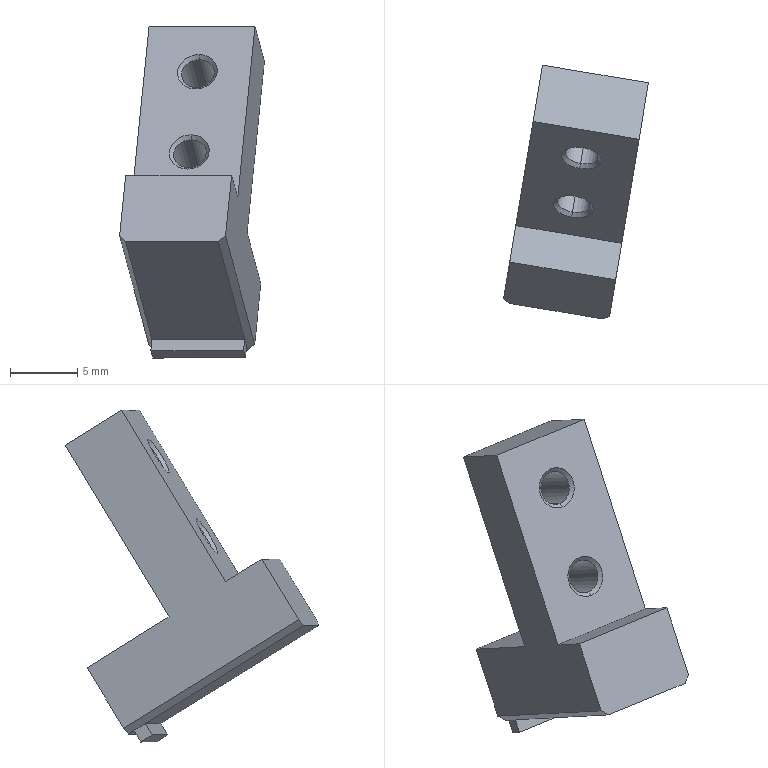Component | SolidWorks | MHZ2_16D_M9BL_14_9_0-1_MHZ2_16D_Finger_0-1 | 1 solid | 30 faces | box 10.79 x 18.88 x 24.73 mm | volume 1274 mm3 | plane 18 | cone 8 | cylinder 4 | commonest cylinder face diameters 2.459 x4
build123d program:
from build123d import *

# Parameters (mm, degrees)
BOSS_EXTRUDE1_DEPTH      = 4
BOSS_EXTRUDE1_DEPTH_BACK = 4
CUT_EXTRUDE1_DEPTH       = 15.5
SKETCH5_W                = 1
SKETCH5_H                = 7
BOSS_EXTRUDE2_DEPTH      = 1


with BuildPart() as part:
    # Sketch1 → Boss-Extrude1 (new, two sides: drawn at the far end of the back side and taken through both)
    with BuildSketch(Plane(origin=(0, 0, 0), x_dir=(1, 0, 0), z_dir=(0, 1, 0)).offset(-BOSS_EXTRUDE1_DEPTH_BACK)):
        Polygon((-18.69, -5.8), (-15.45, -5.8), (-15.45, -20.8), (-10.45, -20.8), (-10.45, -5.8), (-3.19, -5.8), (-3.19, 0), (-18.69, 0), align=None)
    extrude(amount=BOSS_EXTRUDE1_DEPTH + BOSS_EXTRUDE1_DEPTH_BACK)

    # Sketch2 → Cut-Revolve1 (revolve, cut)
    with BuildSketch(Plane(origin=(0, 0, 0), x_dir=(1, 0, 0), z_dir=(0, 1, 0)), mode=Mode.PRIVATE) as cut_revolve1_sk:
        Polygon((-10.45, -16.8), (-10.45, -18.3), (-10.72, -18.029), (-15.18, -18.029), (-15.45, -18.3), (-15.45, -16.8), align=None)
    revolve(cut_revolve1_sk.sketch.rotate(Axis((-15.45, 0, 16.8), (1, 0, 0)), 180), axis=Axis((-15.45, 0, 16.8), (1, 0, 0)), mode=Mode.SUBTRACT)

    # Sketch3 → Cut-Revolve2 (revolve, cut)
    with BuildSketch(Plane(origin=(0, 0, 0), x_dir=(1, 0, 0), z_dir=(0, 1, 0)), mode=Mode.PRIVATE) as cut_revolve2_sk:
        Polygon((-10.45, -9.8), (-10.45, -11.3), (-10.72, -11.03), (-15.18, -11.03), (-15.45, -11.3), (-15.45, -9.8), align=None)
    revolve(cut_revolve2_sk.sketch.rotate(Axis((-15.45, 0, 9.8), (1, 0, 0)), 180), axis=Axis((-15.45, 0, 9.8), (1, 0, 0)), mode=Mode.SUBTRACT)

    # Sketch4 → Cut-Extrude1 (cut)
    with BuildSketch(Plane(origin=(-3.19, 0, 0), x_dir=(0, 0, -1), z_dir=(1, 0, 0))):
        Polygon((-0.5, 4), (0, 3.5), (0, -3.5), (-0.5, -4), (1, -4), (1, 4), align=None)
    extrude(amount=-CUT_EXTRUDE1_DEPTH, mode=Mode.SUBTRACT)

    # Sketch5 → Boss-Extrude2 (add)
    with BuildSketch(Plane(origin=(-3.69, 0, 0), x_dir=(0, 0, -1), z_dir=(1, 0, 0))):
        with Locations((0.5, 0)):
            Rectangle(SKETCH5_W, SKETCH5_H)
    extrude(amount=-BOSS_EXTRUDE2_DEPTH)


solid = part.part

# Placed as in the assembly
solid = solid.moved(Location((525.326, -233.475, -11.504), (-31.129, 4.92, 81.918)))
STEP:
#1=CARTESIAN_POINT('',(20.636,-9.471,0.2295));
#2=VERTEX_POINT('',#1);
#3=CARTESIAN_POINT('',(20.627,-9.521,0.1469));
#4=VERTEX_POINT('',#3);
#5=CARTESIAN_POINT('',(20.631,-9.496,0.1882));
#6=DIRECTION('',(0.1401,0.8413,-0.5222));
#7=DIRECTION('',(-0.08576,-0.5151,-0.8529));
#8=AXIS2_PLACEMENT_3D('',#5,#6,#7);
#9=CIRCLE('',#8,0.04841);
#10=EDGE_CURVE('',#2,#4,#9,.T.);
#11=ORIENTED_EDGE('',*,*,#10,.T.);
#12=CARTESIAN_POINT('',(20.625,-9.535,0.1434));
#13=VERTEX_POINT('',#12);
#14=CARTESIAN_POINT('',(20.625,-9.535,0.1434));
#15=DIRECTION('',(-0.1597,-0.9591,-0.2338));
#16=VECTOR('',#15,39.37);
#17=LINE('',#14,#16);
#18=EDGE_CURVE('',#4,#13,#17,.T.);
#19=ORIENTED_EDGE('',*,*,#18,.T.);
#20=CARTESIAN_POINT('',(20.635,-9.475,0.2441));
#21=VERTEX_POINT('',#20);
#22=CARTESIAN_POINT('',(20.63,-9.505,0.1938));
#23=DIRECTION('',(0.1401,0.8413,-0.5222));
#24=DIRECTION('',(-0.08576,-0.5151,-0.8529));
#25=AXIS2_PLACEMENT_3D('',#22,#23,#24);
#26=CIRCLE('',#25,0.05906);
#27=EDGE_CURVE('',#21,#13,#26,.T.);
#28=ORIENTED_EDGE('',*,*,#27,.F.);
#29=CARTESIAN_POINT('',(20.635,-9.475,0.2441));
#30=DIRECTION('',(-0.03841,-0.2307,0.9723));
#31=VECTOR('',#30,39.37);
#32=LINE('',#29,#31);
#33=EDGE_CURVE('',#2,#21,#32,.T.);
#34=ORIENTED_EDGE('',*,*,#33,.F.);
#35=EDGE_LOOP('',(#11,#19,#28,#34));
#36=FACE_OUTER_BOUND('',#35,.T.);
#37=CARTESIAN_POINT('',(20.63,-9.505,0.1938));
#38=DIRECTION('',(-0.1401,-0.8413,0.5222));
#39=DIRECTION('',(0.08576,0.5151,0.8529));
#40=AXIS2_PLACEMENT_3D('',#37,#38,#39);
#41=CONICAL_SURFACE('',#40,0.05906,0.7854);
#42=ADVANCED_FACE('',(#36),#41,.F.);
#43=ORIENTED_EDGE('',*,*,#10,.F.);
#44=CARTESIAN_POINT('',(20.66,-9.323,0.1378));
#45=VERTEX_POINT('',#44);
#46=CARTESIAN_POINT('',(20.634,-9.48,0.235));
#47=DIRECTION('',(0.1401,0.8413,-0.5222));
#48=VECTOR('',#47,39.37);
#49=LINE('',#46,#48);
#50=EDGE_CURVE('',#2,#45,#49,.T.);
#51=ORIENTED_EDGE('',*,*,#50,.T.);
#52=CARTESIAN_POINT('',(20.652,-9.373,0.05525));
#53=VERTEX_POINT('',#52);
#54=CARTESIAN_POINT('',(20.656,-9.348,0.09653));
#55=DIRECTION('',(0.1401,0.8413,-0.5222));
#56=DIRECTION('',(-0.08576,-0.5151,-0.8529));
#57=AXIS2_PLACEMENT_3D('',#54,#55,#56);
#58=CIRCLE('',#57,0.04841);
#59=EDGE_CURVE('',#45,#53,#58,.T.);
#60=ORIENTED_EDGE('',*,*,#59,.T.);
#61=CARTESIAN_POINT('',(20.626,-9.53,0.1525));
#62=DIRECTION('',(0.1401,0.8413,-0.5222));
#63=VECTOR('',#62,39.37);
#64=LINE('',#61,#63);
#65=EDGE_CURVE('',#4,#53,#64,.T.);
#66=ORIENTED_EDGE('',*,*,#65,.F.);
#67=EDGE_LOOP('',(#43,#51,#60,#66));
#68=FACE_OUTER_BOUND('',#67,.T.);
#69=CARTESIAN_POINT('',(20.63,-9.505,0.1938));
#70=DIRECTION('',(0.1401,0.8413,-0.5222));
#71=DIRECTION('',(-0.08576,-0.5151,-0.8529));
#72=AXIS2_PLACEMENT_3D('',#69,#70,#71);
#73=CYLINDRICAL_SURFACE('',#72,0.04841);
#74=ADVANCED_FACE('',(#68),#73,.F.);
#75=ORIENTED_EDGE('',*,*,#59,.F.);
#76=CARTESIAN_POINT('',(20.663,-9.309,0.1413));
#77=VERTEX_POINT('',#76);
#78=CARTESIAN_POINT('',(20.66,-9.323,0.1378));
#79=DIRECTION('',(0.1597,0.9591,0.2338));
#80=VECTOR('',#79,39.37);
#81=LINE('',#78,#80);
#82=EDGE_CURVE('',#45,#77,#81,.T.);
#83=ORIENTED_EDGE('',*,*,#82,.T.);
#84=CARTESIAN_POINT('',(20.653,-9.37,0.04061));
#85=VERTEX_POINT('',#84);
#86=CARTESIAN_POINT('',(20.658,-9.339,0.09097));
#87=DIRECTION('',(0.1401,0.8413,-0.5222));
#88=DIRECTION('',(-0.08576,-0.5151,-0.8529));
#89=AXIS2_PLACEMENT_3D('',#86,#87,#88);
#90=CIRCLE('',#89,0.05906);
#91=EDGE_CURVE('',#77,#85,#90,.T.);
#92=ORIENTED_EDGE('',*,*,#91,.T.);
#93=CARTESIAN_POINT('',(20.652,-9.373,0.05525));
#94=DIRECTION('',(0.03841,0.2307,-0.9723));
#95=VECTOR('',#94,39.37);
#96=LINE('',#93,#95);
#97=EDGE_CURVE('',#53,#85,#96,.T.);
#98=ORIENTED_EDGE('',*,*,#97,.F.);
#99=EDGE_LOOP('',(#75,#83,#92,#98));
#100=FACE_OUTER_BOUND('',#99,.T.);
#101=CARTESIAN_POINT('',(20.656,-9.348,0.09653));
#102=DIRECTION('',(0.1401,0.8413,-0.5222));
#103=DIRECTION('',(-0.08576,-0.5151,-0.8529));
#104=AXIS2_PLACEMENT_3D('',#101,#102,#103);
#105=CONICAL_SURFACE('',#104,0.04841,0.7854);
#106=ADVANCED_FACE('',(#100),#105,.F.);
#107=CARTESIAN_POINT('',(20.659,-9.329,0.4645));
#108=VERTEX_POINT('',#107);
#109=CARTESIAN_POINT('',(20.651,-9.379,0.382));
#110=VERTEX_POINT('',#109);
#111=CARTESIAN_POINT('',(20.655,-9.354,0.4232));
#112=DIRECTION('',(0.1401,0.8413,-0.5222));
#113=DIRECTION('',(-0.08576,-0.5151,-0.8529));
#114=AXIS2_PLACEMENT_3D('',#111,#112,#113);
#115=CIRCLE('',#114,0.04841);
#116=EDGE_CURVE('',#108,#110,#115,.T.);
#117=ORIENTED_EDGE('',*,*,#116,.T.);
#118=CARTESIAN_POINT('',(20.649,-9.393,0.3784));
#119=VERTEX_POINT('',#118);
#120=CARTESIAN_POINT('',(20.649,-9.393,0.3784));
#121=DIRECTION('',(-0.1597,-0.9591,-0.2338));
#122=VECTOR('',#121,39.37);
#123=LINE('',#120,#122);
#124=EDGE_CURVE('',#110,#119,#123,.T.);
#125=ORIENTED_EDGE('',*,*,#124,.T.);
#126=CARTESIAN_POINT('',(20.659,-9.333,0.4792));
#127=VERTEX_POINT('',#126);
#128=CARTESIAN_POINT('',(20.654,-9.363,0.4288));
#129=DIRECTION('',(0.1401,0.8413,-0.5222));
#130=DIRECTION('',(-0.08576,-0.5151,-0.8529));
#131=AXIS2_PLACEMENT_3D('',#128,#129,#130);
#132=CIRCLE('',#131,0.05906);
#133=EDGE_CURVE('',#127,#119,#132,.T.);
#134=ORIENTED_EDGE('',*,*,#133,.F.);
#135=CARTESIAN_POINT('',(20.659,-9.333,0.4792));
#136=DIRECTION('',(-0.03841,-0.2307,0.9723));
#137=VECTOR('',#136,39.37);
#138=LINE('',#135,#137);
#139=EDGE_CURVE('',#108,#127,#138,.T.);
#140=ORIENTED_EDGE('',*,*,#139,.F.);
#141=EDGE_LOOP('',(#117,#125,#134,#140));
#142=FACE_OUTER_BOUND('',#141,.T.);
#143=CARTESIAN_POINT('',(20.654,-9.363,0.4288));
#144=DIRECTION('',(-0.1401,-0.8413,0.5222));
#145=DIRECTION('',(0.08576,0.5151,0.8529));
#146=AXIS2_PLACEMENT_3D('',#143,#144,#145);
#147=CONICAL_SURFACE('',#146,0.05906,0.7854);
#148=ADVANCED_FACE('',(#142),#147,.F.);
#149=ORIENTED_EDGE('',*,*,#116,.F.);
#150=CARTESIAN_POINT('',(20.684,-9.181,0.3729));
#151=VERTEX_POINT('',#150);
#152=CARTESIAN_POINT('',(20.658,-9.338,0.4701));
#153=DIRECTION('',(0.1401,0.8413,-0.5222));
#154=VECTOR('',#153,39.37);
#155=LINE('',#152,#154);
#156=EDGE_CURVE('',#108,#151,#155,.T.);
#157=ORIENTED_EDGE('',*,*,#156,.T.);
#158=CARTESIAN_POINT('',(20.676,-9.231,0.2903));
#159=VERTEX_POINT('',#158);
#160=CARTESIAN_POINT('',(20.68,-9.206,0.3316));
#161=DIRECTION('',(0.1401,0.8413,-0.5222));
#162=DIRECTION('',(-0.08576,-0.5151,-0.8529));
#163=AXIS2_PLACEMENT_3D('',#160,#161,#162);
#164=CIRCLE('',#163,0.04841);
#165=EDGE_CURVE('',#151,#159,#164,.T.);
#166=ORIENTED_EDGE('',*,*,#165,.T.);
#167=CARTESIAN_POINT('',(20.649,-9.388,0.3875));
#168=DIRECTION('',(0.1401,0.8413,-0.5222));
#169=VECTOR('',#168,39.37);
#170=LINE('',#167,#169);
#171=EDGE_CURVE('',#110,#159,#170,.T.);
#172=ORIENTED_EDGE('',*,*,#171,.F.);
#173=EDGE_LOOP('',(#149,#157,#166,#172));
#174=FACE_OUTER_BOUND('',#173,.T.);
#175=CARTESIAN_POINT('',(20.654,-9.363,0.4288));
#176=DIRECTION('',(0.1401,0.8413,-0.5222));
#177=DIRECTION('',(-0.08576,-0.5151,-0.8529));
#178=AXIS2_PLACEMENT_3D('',#175,#176,#177);
#179=CYLINDRICAL_SURFACE('',#178,0.04841);
#180=ADVANCED_FACE('',(#174),#179,.F.);
#181=ORIENTED_EDGE('',*,*,#165,.F.);
#182=CARTESIAN_POINT('',(20.686,-9.167,0.3764));
#183=VERTEX_POINT('',#182);
#184=CARTESIAN_POINT('',(20.684,-9.181,0.3729));
#185=DIRECTION('',(0.1597,0.9591,0.2338));
#186=VECTOR('',#185,39.37);
#187=LINE('',#184,#186);
#188=EDGE_CURVE('',#151,#183,#187,.T.);
#189=ORIENTED_EDGE('',*,*,#188,.T.);
#190=CARTESIAN_POINT('',(20.676,-9.228,0.2756));
#191=VERTEX_POINT('',#190);
#192=CARTESIAN_POINT('',(20.681,-9.197,0.326));
#193=DIRECTION('',(0.1401,0.8413,-0.5222));
#194=DIRECTION('',(-0.08576,-0.5151,-0.8529));
#195=AXIS2_PLACEMENT_3D('',#192,#193,#194);
#196=CIRCLE('',#195,0.05906);
#197=EDGE_CURVE('',#183,#191,#196,.T.);
#198=ORIENTED_EDGE('',*,*,#197,.T.);
#199=CARTESIAN_POINT('',(20.676,-9.231,0.2903));
#200=DIRECTION('',(0.03841,0.2307,-0.9723));
#201=VECTOR('',#200,39.37);
#202=LINE('',#199,#201);
#203=EDGE_CURVE('',#159,#191,#202,.T.);
#204=ORIENTED_EDGE('',*,*,#203,.F.);
#205=EDGE_LOOP('',(#181,#189,#198,#204));
#206=FACE_OUTER_BOUND('',#205,.T.);
#207=CARTESIAN_POINT('',(20.68,-9.206,0.3316));
#208=DIRECTION('',(0.1401,0.8413,-0.5222));
#209=DIRECTION('',(-0.08576,-0.5151,-0.8529));
#210=AXIS2_PLACEMENT_3D('',#207,#208,#209);
#211=CONICAL_SURFACE('',#210,0.04841,0.7854);
#212=ADVANCED_FACE('',(#206),#211,.F.);
#213=CARTESIAN_POINT('',(20.526,-9.292,-0.377));
#214=VERTEX_POINT('',#213);
#215=CARTESIAN_POINT('',(20.798,-9.337,-0.377));
#216=VERTEX_POINT('',#215);
#217=CARTESIAN_POINT('',(20.526,-9.292,-0.377));
#218=DIRECTION('',(0.9864,-0.1642,0.));
#219=VECTOR('',#218,39.37);
#220=LINE('',#217,#219);
#221=EDGE_CURVE('',#214,#216,#220,.T.);
#222=ORIENTED_EDGE('',*,*,#221,.F.);
#223=CARTESIAN_POINT('',(20.529,-9.275,-0.3873));
#224=VERTEX_POINT('',#223);
#225=CARTESIAN_POINT('',(20.443,-9.788,-0.06869));
#226=DIRECTION('',(0.1401,0.8413,-0.5222));
#227=VECTOR('',#226,39.37);
#228=LINE('',#225,#227);
#229=EDGE_CURVE('',#214,#224,#228,.T.);
#230=ORIENTED_EDGE('',*,*,#229,.T.);
#231=CARTESIAN_POINT('',(20.8,-9.32,-0.3873));
#232=VERTEX_POINT('',#231);
#233=CARTESIAN_POINT('',(20.509,-9.272,-0.3873));
#234=DIRECTION('',(0.9864,-0.1642,0.));
#235=VECTOR('',#234,39.37);
#236=LINE('',#233,#235);
#237=EDGE_CURVE('',#224,#232,#236,.T.);
#238=ORIENTED_EDGE('',*,*,#237,.T.);
#239=CARTESIAN_POINT('',(20.715,-9.834,-0.06869));
#240=DIRECTION('',(0.1401,0.8413,-0.5222));
#241=VECTOR('',#240,39.37);
#242=LINE('',#239,#241);
#243=EDGE_CURVE('',#216,#232,#242,.T.);
#244=ORIENTED_EDGE('',*,*,#243,.F.);
#245=EDGE_LOOP('',(#222,#230,#238,#244));
#246=FACE_OUTER_BOUND('',#245,.T.);
#247=CARTESIAN_POINT('',(20.509,-9.272,-0.3873));
#248=DIRECTION('',(0.08576,0.5151,0.8529));
#249=DIRECTION('',(0.1401,0.8413,-0.5222));
#250=AXIS2_PLACEMENT_3D('',#247,#248,#249);
#251=PLANE('',#250);
#252=ADVANCED_FACE('',(#246),#251,.F.);
#253=CARTESIAN_POINT('',(20.461,-9.56,0.05945));
#254=VERTEX_POINT('',#253);
#255=CARTESIAN_POINT('',(20.772,-9.612,0.05945));
#256=VERTEX_POINT('',#255);
#257=CARTESIAN_POINT('',(20.461,-9.56,0.05945));
#258=DIRECTION('',(0.9864,-0.1642,0.));
#259=VECTOR('',#258,39.37);
#260=LINE('',#257,#259);
#261=EDGE_CURVE('',#254,#256,#260,.T.);
#262=ORIENTED_EDGE('',*,*,#261,.T.);
#263=CARTESIAN_POINT('',(20.822,-9.308,0.5631));
#264=VERTEX_POINT('',#263);
#265=CARTESIAN_POINT('',(20.772,-9.612,0.05945));
#266=DIRECTION('',(0.08576,0.5151,0.8529));
#267=VECTOR('',#266,39.37);
#268=LINE('',#265,#267);
#269=EDGE_CURVE('',#256,#264,#268,.T.);
#270=ORIENTED_EDGE('',*,*,#269,.T.);
#271=CARTESIAN_POINT('',(20.512,-9.256,0.5631));
#272=VERTEX_POINT('',#271);
#273=CARTESIAN_POINT('',(20.512,-9.256,0.5631));
#274=DIRECTION('',(0.9864,-0.1642,0.));
#275=VECTOR('',#274,39.37);
#276=LINE('',#273,#275);
#277=EDGE_CURVE('',#272,#264,#276,.T.);
#278=ORIENTED_EDGE('',*,*,#277,.F.);
#279=CARTESIAN_POINT('',(20.461,-9.56,0.05945));
#280=DIRECTION('',(0.08576,0.5151,0.8529));
#281=VECTOR('',#280,39.37);
#282=LINE('',#279,#281);
#283=EDGE_CURVE('',#254,#272,#282,.T.);
#284=ORIENTED_EDGE('',*,*,#283,.F.);
#285=EDGE_LOOP('',(#262,#270,#278,#284));
#286=FACE_OUTER_BOUND('',#285,.T.);
#287=ORIENTED_EDGE('',*,*,#133,.T.);
#288=CARTESIAN_POINT('',(20.654,-9.363,0.4288));
#289=DIRECTION('',(0.1401,0.8413,-0.5222));
#290=DIRECTION('',(-0.08576,-0.5151,-0.8529));
#291=AXIS2_PLACEMENT_3D('',#288,#289,#290);
#292=CIRCLE('',#291,0.05906);
#293=EDGE_CURVE('',#119,#127,#292,.T.);
#294=ORIENTED_EDGE('',*,*,#293,.T.);
#295=EDGE_LOOP('',(#287,#294));
#296=FACE_BOUND('',#295,.T.);
#297=ORIENTED_EDGE('',*,*,#27,.T.);
#298=CARTESIAN_POINT('',(20.63,-9.505,0.1938));
#299=DIRECTION('',(0.1401,0.8413,-0.5222));
#300=DIRECTION('',(-0.08576,-0.5151,-0.8529));
#301=AXIS2_PLACEMENT_3D('',#298,#299,#300);
#302=CIRCLE('',#301,0.05906);
#303=EDGE_CURVE('',#13,#21,#302,.T.);
#304=ORIENTED_EDGE('',*,*,#303,.T.);
#305=EDGE_LOOP('',(#297,#304));
#306=FACE_BOUND('',#305,.T.);
#307=CARTESIAN_POINT('',(20.461,-9.56,0.05945));
#308=DIRECTION('',(0.1401,0.8413,-0.5222));
#309=DIRECTION('',(-0.08576,-0.5151,-0.8529));
#310=AXIS2_PLACEMENT_3D('',#307,#308,#309);
#311=PLANE('',#310);
#312=ADVANCED_FACE('',(#286,#296,#306),#311,.F.);
#313=CARTESIAN_POINT('',(20.539,-9.09,0.4603));
#314=VERTEX_POINT('',#313);
#315=CARTESIAN_POINT('',(20.85,-9.142,0.4603));
#316=VERTEX_POINT('',#315);
#317=CARTESIAN_POINT('',(20.539,-9.09,0.4603));
#318=DIRECTION('',(0.9864,-0.1642,0.));
#319=VECTOR('',#318,39.37);
#320=LINE('',#317,#319);
#321=EDGE_CURVE('',#314,#316,#320,.T.);
#322=ORIENTED_EDGE('',*,*,#321,.T.);
#323=CARTESIAN_POINT('',(20.799,-9.446,-0.04333));
#324=VERTEX_POINT('',#323);
#325=CARTESIAN_POINT('',(20.85,-9.142,0.4603));
#326=DIRECTION('',(-0.08576,-0.5151,-0.8529));
#327=VECTOR('',#326,39.37);
#328=LINE('',#325,#327);
#329=EDGE_CURVE('',#316,#324,#328,.T.);
#330=ORIENTED_EDGE('',*,*,#329,.T.);
#331=CARTESIAN_POINT('',(20.489,-9.395,-0.04333));
#332=VERTEX_POINT('',#331);
#333=CARTESIAN_POINT('',(20.489,-9.395,-0.04333));
#334=DIRECTION('',(0.9864,-0.1642,0.));
#335=VECTOR('',#334,39.37);
#336=LINE('',#333,#335);
#337=EDGE_CURVE('',#332,#324,#336,.T.);
#338=ORIENTED_EDGE('',*,*,#337,.F.);
#339=CARTESIAN_POINT('',(20.539,-9.09,0.4603));
#340=DIRECTION('',(-0.08576,-0.5151,-0.8529));
#341=VECTOR('',#340,39.37);
#342=LINE('',#339,#341);
#343=EDGE_CURVE('',#314,#332,#342,.T.);
#344=ORIENTED_EDGE('',*,*,#343,.F.);
#345=EDGE_LOOP('',(#322,#330,#338,#344));
#346=FACE_OUTER_BOUND('',#345,.T.);
#347=CARTESIAN_POINT('',(20.681,-9.197,0.326));
#348=DIRECTION('',(0.1401,0.8413,-0.5222));
#349=DIRECTION('',(-0.08576,-0.5151,-0.8529));
#350=AXIS2_PLACEMENT_3D('',#347,#348,#349);
#351=CIRCLE('',#350,0.05906);
#352=EDGE_CURVE('',#191,#183,#351,.T.);
#353=ORIENTED_EDGE('',*,*,#352,.F.);
#354=ORIENTED_EDGE('',*,*,#197,.F.);
#355=EDGE_LOOP('',(#353,#354));
#356=FACE_BOUND('',#355,.T.);
#357=CARTESIAN_POINT('',(20.658,-9.339,0.09097));
#358=DIRECTION('',(0.1401,0.8413,-0.5222));
#359=DIRECTION('',(-0.08576,-0.5151,-0.8529));
#360=AXIS2_PLACEMENT_3D('',#357,#358,#359);
#361=CIRCLE('',#360,0.05906);
#362=EDGE_CURVE('',#85,#77,#361,.T.);
#363=ORIENTED_EDGE('',*,*,#362,.F.);
#364=ORIENTED_EDGE('',*,*,#91,.F.);
#365=EDGE_LOOP('',(#363,#364));
#366=FACE_BOUND('',#365,.T.);
#367=CARTESIAN_POINT('',(20.539,-9.09,0.4603));
#368=DIRECTION('',(-0.1401,-0.8413,0.5222));
#369=DIRECTION('',(0.08576,0.5151,0.8529));
#370=AXIS2_PLACEMENT_3D('',#367,#368,#369);
#371=PLANE('',#370);
#372=ADVANCED_FACE('',(#346,#356,#366),#371,.F.);
#373=CARTESIAN_POINT('',(20.443,-9.788,-0.06869));
#374=VERTEX_POINT('',#373);
#375=CARTESIAN_POINT('',(20.715,-9.834,-0.06869));
#376=VERTEX_POINT('',#375);
#377=CARTESIAN_POINT('',(20.424,-9.785,-0.06869));
#378=DIRECTION('',(0.9864,-0.1642,0.));
#379=VECTOR('',#378,39.37);
#380=LINE('',#377,#379);
#381=EDGE_CURVE('',#374,#376,#380,.T.);
#382=ORIENTED_EDGE('',*,*,#381,.T.);
#383=CARTESIAN_POINT('',(20.736,-9.827,-0.0519));
#384=VERTEX_POINT('',#383);
#385=CARTESIAN_POINT('',(20.715,-9.834,-0.06869));
#386=DIRECTION('',(0.7581,0.2481,0.6031));
#387=VECTOR('',#386,39.37);
#388=LINE('',#385,#387);
#389=EDGE_CURVE('',#376,#384,#388,.T.);
#390=ORIENTED_EDGE('',*,*,#389,.T.);
#391=CARTESIAN_POINT('',(20.754,-9.719,0.1261));
#392=VERTEX_POINT('',#391);
#393=CARTESIAN_POINT('',(20.734,-9.837,-0.06869));
#394=DIRECTION('',(0.08576,0.5151,0.8529));
#395=VECTOR('',#394,39.37);
#396=LINE('',#393,#395);
#397=EDGE_CURVE('',#384,#392,#396,.T.);
#398=ORIENTED_EDGE('',*,*,#397,.T.);
#399=CARTESIAN_POINT('',(20.443,-9.667,0.1261));
#400=VERTEX_POINT('',#399);
#401=CARTESIAN_POINT('',(20.443,-9.667,0.1261));
#402=DIRECTION('',(0.9864,-0.1642,0.));
#403=VECTOR('',#402,39.37);
#404=LINE('',#401,#403);
#405=EDGE_CURVE('',#400,#392,#404,.T.);
#406=ORIENTED_EDGE('',*,*,#405,.F.);
#407=CARTESIAN_POINT('',(20.425,-9.775,-0.0519));
#408=VERTEX_POINT('',#407);
#409=CARTESIAN_POINT('',(20.424,-9.785,-0.06869));
#410=DIRECTION('',(0.08576,0.5151,0.8529));
#411=VECTOR('',#410,39.37);
#412=LINE('',#409,#411);
#413=EDGE_CURVE('',#408,#400,#412,.T.);
#414=ORIENTED_EDGE('',*,*,#413,.F.);
#415=CARTESIAN_POINT('',(20.425,-9.775,-0.0519));
#416=DIRECTION('',(0.6369,-0.4803,-0.6031));
#417=VECTOR('',#416,39.37);
#418=LINE('',#415,#417);
#419=EDGE_CURVE('',#408,#374,#418,.T.);
#420=ORIENTED_EDGE('',*,*,#419,.T.);
#421=EDGE_LOOP('',(#382,#390,#398,#406,#414,#420));
#422=FACE_OUTER_BOUND('',#421,.T.);
#423=CARTESIAN_POINT('',(20.424,-9.785,-0.06869));
#424=DIRECTION('',(0.1401,0.8413,-0.5222));
#425=DIRECTION('',(-0.08576,-0.5151,-0.8529));
#426=AXIS2_PLACEMENT_3D('',#423,#424,#425);
#427=PLANE('',#426);
#428=ADVANCED_FACE('',(#422),#427,.F.);
#429=ORIENTED_EDGE('',*,*,#405,.T.);
#430=CARTESIAN_POINT('',(20.754,-9.719,0.1261));
#431=DIRECTION('',(0.1401,0.8413,-0.5222));
#432=VECTOR('',#431,39.37);
#433=LINE('',#430,#432);
#434=EDGE_CURVE('',#392,#256,#433,.T.);
#435=ORIENTED_EDGE('',*,*,#434,.T.);
#436=ORIENTED_EDGE('',*,*,#261,.F.);
#437=CARTESIAN_POINT('',(20.443,-9.667,0.1261));
#438=DIRECTION('',(0.1401,0.8413,-0.5222));
#439=VECTOR('',#438,39.37);
#440=LINE('',#437,#439);
#441=EDGE_CURVE('',#400,#254,#440,.T.);
#442=ORIENTED_EDGE('',*,*,#441,.F.);
#443=EDGE_LOOP('',(#429,#435,#436,#442));
#444=FACE_OUTER_BOUND('',#443,.T.);
#445=CARTESIAN_POINT('',(20.443,-9.667,0.1261));
#446=DIRECTION('',(-0.08576,-0.5151,-0.8529));
#447=DIRECTION('',(-0.1401,-0.8413,0.5222));
#448=AXIS2_PLACEMENT_3D('',#445,#446,#447);
#449=PLANE('',#448);
#450=ADVANCED_FACE('',(#444),#449,.F.);
#451=ORIENTED_EDGE('',*,*,#277,.T.);
#452=CARTESIAN_POINT('',(20.822,-9.308,0.5631));
#453=DIRECTION('',(0.1401,0.8413,-0.5222));
#454=VECTOR('',#453,39.37);
#455=LINE('',#452,#454);
#456=EDGE_CURVE('',#264,#316,#455,.T.);
#457=ORIENTED_EDGE('',*,*,#456,.T.);
#458=ORIENTED_EDGE('',*,*,#321,.F.);
#459=CARTESIAN_POINT('',(20.512,-9.256,0.5631));
#460=DIRECTION('',(0.1401,0.8413,-0.5222));
#461=VECTOR('',#460,39.37);
#462=LINE('',#459,#461);
#463=EDGE_CURVE('',#272,#314,#462,.T.);
#464=ORIENTED_EDGE('',*,*,#463,.F.);
#465=EDGE_LOOP('',(#451,#457,#458,#464));
#466=FACE_OUTER_BOUND('',#465,.T.);
#467=CARTESIAN_POINT('',(20.512,-9.256,0.5631));
#468=DIRECTION('',(-0.08576,-0.5151,-0.8529));
#469=DIRECTION('',(-0.1401,-0.8413,0.5222));
#470=AXIS2_PLACEMENT_3D('',#467,#468,#469);
#471=PLANE('',#470);
#472=ADVANCED_FACE('',(#466),#471,.F.);
#473=ORIENTED_EDGE('',*,*,#337,.T.);
#474=CARTESIAN_POINT('',(20.839,-9.206,-0.1926));
#475=VERTEX_POINT('',#474);
#476=CARTESIAN_POINT('',(20.799,-9.446,-0.04333));
#477=DIRECTION('',(0.1401,0.8413,-0.5222));
#478=VECTOR('',#477,39.37);
#479=LINE('',#476,#478);
#480=EDGE_CURVE('',#324,#475,#479,.T.);
#481=ORIENTED_EDGE('',*,*,#480,.T.);
#482=CARTESIAN_POINT('',(20.529,-9.154,-0.1926));
#483=VERTEX_POINT('',#482);
#484=CARTESIAN_POINT('',(20.529,-9.154,-0.1926));
#485=DIRECTION('',(0.9864,-0.1642,0.));
#486=VECTOR('',#485,39.37);
#487=LINE('',#484,#486);
#488=EDGE_CURVE('',#483,#475,#487,.T.);
#489=ORIENTED_EDGE('',*,*,#488,.F.);
#490=CARTESIAN_POINT('',(20.489,-9.395,-0.04333));
#491=DIRECTION('',(0.1401,0.8413,-0.5222));
#492=VECTOR('',#491,39.37);
#493=LINE('',#490,#492);
#494=EDGE_CURVE('',#332,#483,#493,.T.);
#495=ORIENTED_EDGE('',*,*,#494,.F.);
#496=EDGE_LOOP('',(#473,#481,#489,#495));
#497=FACE_OUTER_BOUND('',#496,.T.);
#498=CARTESIAN_POINT('',(20.489,-9.395,-0.04333));
#499=DIRECTION('',(-0.08576,-0.5151,-0.8529));
#500=DIRECTION('',(-0.1401,-0.8413,0.5222));
#501=AXIS2_PLACEMENT_3D('',#498,#499,#500);
#502=PLANE('',#501);
#503=ADVANCED_FACE('',(#497),#502,.F.);
#504=CARTESIAN_POINT('',(20.822,-9.313,-0.3705));
#505=VERTEX_POINT('',#504);
#506=CARTESIAN_POINT('',(20.839,-9.206,-0.1926));
#507=DIRECTION('',(-0.08576,-0.5151,-0.8529));
#508=VECTOR('',#507,39.37);
#509=LINE('',#506,#508);
#510=EDGE_CURVE('',#475,#505,#509,.T.);
#511=ORIENTED_EDGE('',*,*,#510,.T.);
#512=CARTESIAN_POINT('',(20.8,-9.32,-0.3873));
#513=DIRECTION('',(0.7581,0.2481,0.6031));
#514=VECTOR('',#513,39.37);
#515=LINE('',#512,#514);
#516=EDGE_CURVE('',#232,#505,#515,.T.);
#517=ORIENTED_EDGE('',*,*,#516,.F.);
#518=ORIENTED_EDGE('',*,*,#237,.F.);
#519=CARTESIAN_POINT('',(20.511,-9.262,-0.3705));
#520=VERTEX_POINT('',#519);
#521=CARTESIAN_POINT('',(20.511,-9.262,-0.3705));
#522=DIRECTION('',(0.6369,-0.4803,-0.6031));
#523=VECTOR('',#522,39.37);
#524=LINE('',#521,#523);
#525=EDGE_CURVE('',#520,#224,#524,.T.);
#526=ORIENTED_EDGE('',*,*,#525,.F.);
#527=CARTESIAN_POINT('',(20.529,-9.154,-0.1926));
#528=DIRECTION('',(-0.08576,-0.5151,-0.8529));
#529=VECTOR('',#528,39.37);
#530=LINE('',#527,#529);
#531=EDGE_CURVE('',#483,#520,#530,.T.);
#532=ORIENTED_EDGE('',*,*,#531,.F.);
#533=ORIENTED_EDGE('',*,*,#488,.T.);
#534=EDGE_LOOP('',(#511,#517,#518,#526,#532,#533));
#535=FACE_OUTER_BOUND('',#534,.T.);
#536=CARTESIAN_POINT('',(20.529,-9.154,-0.1926));
#537=DIRECTION('',(-0.1401,-0.8413,0.5222));
#538=DIRECTION('',(0.08576,0.5151,0.8529));
#539=AXIS2_PLACEMENT_3D('',#536,#537,#538);
#540=PLANE('',#539);
#541=ADVANCED_FACE('',(#535),#540,.F.);
#542=CARTESIAN_POINT('',(20.52,-9.325,-0.3565));
#543=VERTEX_POINT('',#542);
#544=CARTESIAN_POINT('',(20.443,-9.788,-0.06869));
#545=DIRECTION('',(0.1401,0.8413,-0.5222));
#546=VECTOR('',#545,39.37);
#547=LINE('',#544,#546);
#548=EDGE_CURVE('',#374,#543,#547,.T.);
#549=ORIENTED_EDGE('',*,*,#548,.T.);
#550=CARTESIAN_POINT('',(20.792,-9.37,-0.3565));
#551=VERTEX_POINT('',#550);
#552=CARTESIAN_POINT('',(20.52,-9.325,-0.3565));
#553=DIRECTION('',(0.9864,-0.1642,0.));
#554=VECTOR('',#553,39.37);
#555=LINE('',#552,#554);
#556=EDGE_CURVE('',#543,#551,#555,.T.);
#557=ORIENTED_EDGE('',*,*,#556,.T.);
#558=CARTESIAN_POINT('',(20.715,-9.834,-0.06869));
#559=DIRECTION('',(0.1401,0.8413,-0.5222));
#560=VECTOR('',#559,39.37);
#561=LINE('',#558,#560);
#562=EDGE_CURVE('',#376,#551,#561,.T.);
#563=ORIENTED_EDGE('',*,*,#562,.F.);
#564=ORIENTED_EDGE('',*,*,#381,.F.);
#565=EDGE_LOOP('',(#549,#557,#563,#564));
#566=FACE_OUTER_BOUND('',#565,.T.);
#567=CARTESIAN_POINT('',(20.509,-9.272,-0.3873));
#568=DIRECTION('',(0.08576,0.5151,0.8529));
#569=DIRECTION('',(0.1401,0.8413,-0.5222));
#570=AXIS2_PLACEMENT_3D('',#567,#568,#569);
#571=PLANE('',#570);
#572=ADVANCED_FACE('',(#566),#571,.F.);
#573=CARTESIAN_POINT('',(20.425,-9.775,-0.0519));
#574=DIRECTION('',(0.1401,0.8413,-0.5222));
#575=VECTOR('',#574,39.37);
#576=LINE('',#573,#575);
#577=EDGE_CURVE('',#408,#520,#576,.T.);
#578=ORIENTED_EDGE('',*,*,#577,.F.);
#579=ORIENTED_EDGE('',*,*,#413,.T.);
#580=ORIENTED_EDGE('',*,*,#441,.T.);
#581=ORIENTED_EDGE('',*,*,#283,.T.);
#582=ORIENTED_EDGE('',*,*,#463,.T.);
#583=ORIENTED_EDGE('',*,*,#343,.T.);
#584=ORIENTED_EDGE('',*,*,#494,.T.);
#585=ORIENTED_EDGE('',*,*,#531,.T.);
#586=EDGE_LOOP('',(#578,#579,#580,#581,#582,#583,#584,#585));
#587=FACE_OUTER_BOUND('',#586,.T.);
#588=CARTESIAN_POINT('',(20.527,-9.166,-0.4529));
#589=DIRECTION('',(-0.9864,0.1642,-0.));
#590=DIRECTION('',(0.08576,0.5151,0.8529));
#591=AXIS2_PLACEMENT_3D('',#588,#589,#590);
#592=PLANE('',#591);
#593=ADVANCED_FACE('',(#587),#592,.T.);
#594=ORIENTED_EDGE('',*,*,#397,.F.);
#595=CARTESIAN_POINT('',(20.736,-9.827,-0.0519));
#596=DIRECTION('',(0.1401,0.8413,-0.5222));
#597=VECTOR('',#596,39.37);
#598=LINE('',#595,#597);
#599=EDGE_CURVE('',#384,#505,#598,.T.);
#600=ORIENTED_EDGE('',*,*,#599,.T.);
#601=ORIENTED_EDGE('',*,*,#510,.F.);
#602=ORIENTED_EDGE('',*,*,#480,.F.);
#603=ORIENTED_EDGE('',*,*,#329,.F.);
#604=ORIENTED_EDGE('',*,*,#456,.F.);
#605=ORIENTED_EDGE('',*,*,#269,.F.);
#606=ORIENTED_EDGE('',*,*,#434,.F.);
#607=EDGE_LOOP('',(#594,#600,#601,#602,#603,#604,#605,#606));
#608=FACE_OUTER_BOUND('',#607,.T.);
#609=CARTESIAN_POINT('',(20.837,-9.218,-0.4529));
#610=DIRECTION('',(-0.9864,0.1642,-0.));
#611=DIRECTION('',(0.08576,0.5151,0.8529));
#612=AXIS2_PLACEMENT_3D('',#609,#610,#611);
#613=PLANE('',#612);
#614=ADVANCED_FACE('',(#608),#613,.F.);
#615=ORIENTED_EDGE('',*,*,#188,.F.);
#616=CARTESIAN_POINT('',(20.68,-9.206,0.3316));
#617=DIRECTION('',(0.1401,0.8413,-0.5222));
#618=DIRECTION('',(-0.08576,-0.5151,-0.8529));
#619=AXIS2_PLACEMENT_3D('',#616,#617,#618);
#620=CIRCLE('',#619,0.04841);
#621=EDGE_CURVE('',#159,#151,#620,.T.);
#622=ORIENTED_EDGE('',*,*,#621,.F.);
#623=ORIENTED_EDGE('',*,*,#203,.T.);
#624=ORIENTED_EDGE('',*,*,#352,.T.);
#625=EDGE_LOOP('',(#615,#622,#623,#624));
#626=FACE_OUTER_BOUND('',#625,.T.);
#627=CARTESIAN_POINT('',(20.68,-9.206,0.3316));
#628=DIRECTION('',(0.1401,0.8413,-0.5222));
#629=DIRECTION('',(-0.08576,-0.5151,-0.8529));
#630=AXIS2_PLACEMENT_3D('',#627,#628,#629);
#631=CONICAL_SURFACE('',#630,0.04841,0.7854);
#632=ADVANCED_FACE('',(#626),#631,.F.);
#633=ORIENTED_EDGE('',*,*,#156,.F.);
#634=CARTESIAN_POINT('',(20.655,-9.354,0.4232));
#635=DIRECTION('',(0.1401,0.8413,-0.5222));
#636=DIRECTION('',(-0.08576,-0.5151,-0.8529));
#637=AXIS2_PLACEMENT_3D('',#634,#635,#636);
#638=CIRCLE('',#637,0.04841);
#639=EDGE_CURVE('',#110,#108,#638,.T.);
#640=ORIENTED_EDGE('',*,*,#639,.F.);
#641=ORIENTED_EDGE('',*,*,#171,.T.);
#642=ORIENTED_EDGE('',*,*,#621,.T.);
#643=EDGE_LOOP('',(#633,#640,#641,#642));
#644=FACE_OUTER_BOUND('',#643,.T.);
#645=CARTESIAN_POINT('',(20.654,-9.363,0.4288));
#646=DIRECTION('',(0.1401,0.8413,-0.5222));
#647=DIRECTION('',(-0.08576,-0.5151,-0.8529));
#648=AXIS2_PLACEMENT_3D('',#645,#646,#647);
#649=CYLINDRICAL_SURFACE('',#648,0.04841);
#650=ADVANCED_FACE('',(#644),#649,.F.);
#651=ORIENTED_EDGE('',*,*,#124,.F.);
#652=ORIENTED_EDGE('',*,*,#639,.T.);
#653=ORIENTED_EDGE('',*,*,#139,.T.);
#654=ORIENTED_EDGE('',*,*,#293,.F.);
#655=EDGE_LOOP('',(#651,#652,#653,#654));
#656=FACE_OUTER_BOUND('',#655,.T.);
#657=CARTESIAN_POINT('',(20.654,-9.363,0.4288));
#658=DIRECTION('',(-0.1401,-0.8413,0.5222));
#659=DIRECTION('',(0.08576,0.5151,0.8529));
#660=AXIS2_PLACEMENT_3D('',#657,#658,#659);
#661=CONICAL_SURFACE('',#660,0.05906,0.7854);
#662=ADVANCED_FACE('',(#656),#661,.F.);
#663=ORIENTED_EDGE('',*,*,#82,.F.);
#664=CARTESIAN_POINT('',(20.656,-9.348,0.09653));
#665=DIRECTION('',(0.1401,0.8413,-0.5222));
#666=DIRECTION('',(-0.08576,-0.5151,-0.8529));
#667=AXIS2_PLACEMENT_3D('',#664,#665,#666);
#668=CIRCLE('',#667,0.04841);
#669=EDGE_CURVE('',#53,#45,#668,.T.);
#670=ORIENTED_EDGE('',*,*,#669,.F.);
#671=ORIENTED_EDGE('',*,*,#97,.T.);
#672=ORIENTED_EDGE('',*,*,#362,.T.);
#673=EDGE_LOOP('',(#663,#670,#671,#672));
#674=FACE_OUTER_BOUND('',#673,.T.);
#675=CARTESIAN_POINT('',(20.656,-9.348,0.09653));
#676=DIRECTION('',(0.1401,0.8413,-0.5222));
#677=DIRECTION('',(-0.08576,-0.5151,-0.8529));
#678=AXIS2_PLACEMENT_3D('',#675,#676,#677);
#679=CONICAL_SURFACE('',#678,0.04841,0.7854);
#680=ADVANCED_FACE('',(#674),#679,.F.);
#681=ORIENTED_EDGE('',*,*,#50,.F.);
#682=CARTESIAN_POINT('',(20.631,-9.496,0.1882));
#683=DIRECTION('',(0.1401,0.8413,-0.5222));
#684=DIRECTION('',(-0.08576,-0.5151,-0.8529));
#685=AXIS2_PLACEMENT_3D('',#682,#683,#684);
#686=CIRCLE('',#685,0.04841);
#687=EDGE_CURVE('',#4,#2,#686,.T.);
#688=ORIENTED_EDGE('',*,*,#687,.F.);
#689=ORIENTED_EDGE('',*,*,#65,.T.);
#690=ORIENTED_EDGE('',*,*,#669,.T.);
#691=EDGE_LOOP('',(#681,#688,#689,#690));
#692=FACE_OUTER_BOUND('',#691,.T.);
#693=CARTESIAN_POINT('',(20.63,-9.505,0.1938));
#694=DIRECTION('',(0.1401,0.8413,-0.5222));
#695=DIRECTION('',(-0.08576,-0.5151,-0.8529));
#696=AXIS2_PLACEMENT_3D('',#693,#694,#695);
#697=CYLINDRICAL_SURFACE('',#696,0.04841);
#698=ADVANCED_FACE('',(#692),#697,.F.);
#699=ORIENTED_EDGE('',*,*,#18,.F.);
#700=ORIENTED_EDGE('',*,*,#687,.T.);
#701=ORIENTED_EDGE('',*,*,#33,.T.);
#702=ORIENTED_EDGE('',*,*,#303,.F.);
#703=EDGE_LOOP('',(#699,#700,#701,#702));
#704=FACE_OUTER_BOUND('',#703,.T.);
#705=CARTESIAN_POINT('',(20.63,-9.505,0.1938));
#706=DIRECTION('',(-0.1401,-0.8413,0.5222));
#707=DIRECTION('',(0.08576,0.5151,0.8529));
#708=AXIS2_PLACEMENT_3D('',#705,#706,#707);
#709=CONICAL_SURFACE('',#708,0.05906,0.7854);
#710=ADVANCED_FACE('',(#704),#709,.F.);
#711=ORIENTED_EDGE('',*,*,#516,.T.);
#712=ORIENTED_EDGE('',*,*,#599,.F.);
#713=ORIENTED_EDGE('',*,*,#389,.F.);
#714=ORIENTED_EDGE('',*,*,#562,.T.);
#715=CARTESIAN_POINT('',(20.792,-9.37,-0.3565));
#716=DIRECTION('',(0.1401,0.8413,-0.5222));
#717=VECTOR('',#716,39.37);
#718=LINE('',#715,#717);
#719=EDGE_CURVE('',#551,#216,#718,.T.);
#720=ORIENTED_EDGE('',*,*,#719,.T.);
#721=ORIENTED_EDGE('',*,*,#243,.T.);
#722=EDGE_LOOP('',(#711,#712,#713,#714,#720,#721));
#723=FACE_OUTER_BOUND('',#722,.T.);
#724=CARTESIAN_POINT('',(20.715,-9.834,-0.06869));
#725=DIRECTION('',(-0.6369,0.4803,0.6031));
#726=DIRECTION('',(0.7581,0.2481,0.6031));
#727=AXIS2_PLACEMENT_3D('',#724,#725,#726);
#728=PLANE('',#727);
#729=ADVANCED_FACE('',(#723),#728,.F.);
#730=ORIENTED_EDGE('',*,*,#525,.T.);
#731=ORIENTED_EDGE('',*,*,#229,.F.);
#732=CARTESIAN_POINT('',(20.52,-9.325,-0.3565));
#733=DIRECTION('',(0.1401,0.8413,-0.5222));
#734=VECTOR('',#733,39.37);
#735=LINE('',#732,#734);
#736=EDGE_CURVE('',#543,#214,#735,.T.);
#737=ORIENTED_EDGE('',*,*,#736,.F.);
#738=ORIENTED_EDGE('',*,*,#548,.F.);
#739=ORIENTED_EDGE('',*,*,#419,.F.);
#740=ORIENTED_EDGE('',*,*,#577,.T.);
#741=EDGE_LOOP('',(#730,#731,#737,#738,#739,#740));
#742=FACE_OUTER_BOUND('',#741,.T.);
#743=CARTESIAN_POINT('',(20.425,-9.775,-0.0519));
#744=DIRECTION('',(0.7581,0.2481,0.6031));
#745=DIRECTION('',(0.6369,-0.4803,-0.6031));
#746=AXIS2_PLACEMENT_3D('',#743,#744,#745);
#747=PLANE('',#746);
#748=ADVANCED_FACE('',(#742),#747,.F.);
#749=CARTESIAN_POINT('',(20.522,-9.312,-0.4106));
#750=VERTEX_POINT('',#749);
#751=CARTESIAN_POINT('',(20.522,-9.312,-0.4106));
#752=DIRECTION('',(0.08576,0.5151,0.8529));
#753=VECTOR('',#752,39.37);
#754=LINE('',#751,#753);
#755=EDGE_CURVE('',#750,#214,#754,.T.);
#756=ORIENTED_EDGE('',*,*,#755,.F.);
#757=CARTESIAN_POINT('',(20.517,-9.345,-0.3901));
#758=VERTEX_POINT('',#757);
#759=CARTESIAN_POINT('',(20.517,-9.345,-0.3901));
#760=DIRECTION('',(0.1401,0.8413,-0.5222));
#761=VECTOR('',#760,39.37);
#762=LINE('',#759,#761);
#763=EDGE_CURVE('',#758,#750,#762,.T.);
#764=ORIENTED_EDGE('',*,*,#763,.F.);
#765=CARTESIAN_POINT('',(20.517,-9.345,-0.3901));
#766=DIRECTION('',(0.08576,0.5151,0.8529));
#767=VECTOR('',#766,39.37);
#768=LINE('',#765,#767);
#769=EDGE_CURVE('',#758,#543,#768,.T.);
#770=ORIENTED_EDGE('',*,*,#769,.T.);
#771=ORIENTED_EDGE('',*,*,#736,.T.);
#772=EDGE_LOOP('',(#756,#764,#770,#771));
#773=FACE_OUTER_BOUND('',#772,.T.);
#774=CARTESIAN_POINT('',(20.517,-9.345,-0.3901));
#775=DIRECTION('',(-0.9864,0.1642,-0.));
#776=DIRECTION('',(0.08576,0.5151,0.8529));
#777=AXIS2_PLACEMENT_3D('',#774,#775,#776);
#778=PLANE('',#777);
#779=ADVANCED_FACE('',(#773),#778,.T.);
#780=CARTESIAN_POINT('',(20.794,-9.357,-0.4106));
#781=VERTEX_POINT('',#780);
#782=CARTESIAN_POINT('',(20.794,-9.357,-0.4106));
#783=DIRECTION('',(-0.9864,0.1642,-0.));
#784=VECTOR('',#783,39.37);
#785=LINE('',#782,#784);
#786=EDGE_CURVE('',#781,#750,#785,.T.);
#787=ORIENTED_EDGE('',*,*,#786,.F.);
#788=CARTESIAN_POINT('',(20.789,-9.39,-0.3901));
#789=VERTEX_POINT('',#788);
#790=CARTESIAN_POINT('',(20.789,-9.39,-0.3901));
#791=DIRECTION('',(0.1401,0.8413,-0.5222));
#792=VECTOR('',#791,39.37);
#793=LINE('',#790,#792);
#794=EDGE_CURVE('',#789,#781,#793,.T.);
#795=ORIENTED_EDGE('',*,*,#794,.F.);
#796=CARTESIAN_POINT('',(20.789,-9.39,-0.3901));
#797=DIRECTION('',(-0.9864,0.1642,-0.));
#798=VECTOR('',#797,39.37);
#799=LINE('',#796,#798);
#800=EDGE_CURVE('',#789,#758,#799,.T.);
#801=ORIENTED_EDGE('',*,*,#800,.T.);
#802=ORIENTED_EDGE('',*,*,#763,.T.);
#803=EDGE_LOOP('',(#787,#795,#801,#802));
#804=FACE_OUTER_BOUND('',#803,.T.);
#805=CARTESIAN_POINT('',(20.789,-9.39,-0.3901));
#806=DIRECTION('',(-0.08576,-0.5151,-0.8529));
#807=DIRECTION('',(-0.1401,-0.8413,0.5222));
#808=AXIS2_PLACEMENT_3D('',#805,#806,#807);
#809=PLANE('',#808);
#810=ADVANCED_FACE('',(#804),#809,.T.);
#811=CARTESIAN_POINT('',(20.798,-9.337,-0.377));
#812=DIRECTION('',(-0.08576,-0.5151,-0.8529));
#813=VECTOR('',#812,39.37);
#814=LINE('',#811,#813);
#815=EDGE_CURVE('',#216,#781,#814,.T.);
#816=ORIENTED_EDGE('',*,*,#815,.F.);
#817=ORIENTED_EDGE('',*,*,#719,.F.);
#818=CARTESIAN_POINT('',(20.792,-9.37,-0.3565));
#819=DIRECTION('',(-0.08576,-0.5151,-0.8529));
#820=VECTOR('',#819,39.37);
#821=LINE('',#818,#820);
#822=EDGE_CURVE('',#551,#789,#821,.T.);
#823=ORIENTED_EDGE('',*,*,#822,.T.);
#824=ORIENTED_EDGE('',*,*,#794,.T.);
#825=EDGE_LOOP('',(#816,#817,#823,#824));
#826=FACE_OUTER_BOUND('',#825,.T.);
#827=CARTESIAN_POINT('',(20.792,-9.37,-0.3565));
#828=DIRECTION('',(0.9864,-0.1642,0.));
#829=DIRECTION('',(-0.08576,-0.5151,-0.8529));
#830=AXIS2_PLACEMENT_3D('',#827,#828,#829);
#831=PLANE('',#830);
#832=ADVANCED_FACE('',(#826),#831,.T.);
#833=ORIENTED_EDGE('',*,*,#556,.F.);
#834=ORIENTED_EDGE('',*,*,#769,.F.);
#835=ORIENTED_EDGE('',*,*,#800,.F.);
#836=ORIENTED_EDGE('',*,*,#822,.F.);
#837=EDGE_LOOP('',(#833,#834,#835,#836));
#838=FACE_OUTER_BOUND('',#837,.T.);
#839=CARTESIAN_POINT('',(20.656,-9.347,-0.3565));
#840=DIRECTION('',(0.1401,0.8413,-0.5222));
#841=DIRECTION('',(-0.08576,-0.5151,-0.8529));
#842=AXIS2_PLACEMENT_3D('',#839,#840,#841);
#843=PLANE('',#842);
#844=ADVANCED_FACE('',(#838),#843,.F.);
#845=ORIENTED_EDGE('',*,*,#221,.T.);
#846=ORIENTED_EDGE('',*,*,#815,.T.);
#847=ORIENTED_EDGE('',*,*,#786,.T.);
#848=ORIENTED_EDGE('',*,*,#755,.T.);
#849=EDGE_LOOP('',(#845,#846,#847,#848));
#850=FACE_OUTER_BOUND('',#849,.T.);
#851=CARTESIAN_POINT('',(20.662,-9.314,-0.377));
#852=DIRECTION('',(0.1401,0.8413,-0.5222));
#853=DIRECTION('',(-0.08576,-0.5151,-0.8529));
#854=AXIS2_PLACEMENT_3D('',#851,#852,#853);
#855=PLANE('',#854);
#856=ADVANCED_FACE('',(#850),#855,.T.);
#857=CLOSED_SHELL('',(#42,#74,#106,#148,#180,#212,#252,#312,#372,#428,#450,#472,#503,#541,#572,#593,#614,#632,#650,#662,#680,#698,#710,#729,#748,#779,#810,#832,#844,#856));
#858=MANIFOLD_SOLID_BREP('',#857);
#859=CARTESIAN_POINT('',(0.,0.,0.));
#860=DIRECTION('',(0.,0.,1.));
#861=DIRECTION('',(1.,0.,0.));
#862=AXIS2_PLACEMENT_3D('',#859,#860,#861);
#863=(LENGTH_UNIT()NAMED_UNIT(*)SI_UNIT($,.METRE.));
#864=LENGTH_MEASURE_WITH_UNIT(LENGTH_MEASURE(0.0254),#863);
#865=DIMENSIONAL_EXPONENTS(1.,0.,0.,0.,0.,0.,0.);
#866=(CONVERSION_BASED_UNIT('',#864)LENGTH_UNIT()NAMED_UNIT(#865));
#867=UNCERTAINTY_MEASURE_WITH_UNIT(LENGTH_MEASURE(0.00001),#866,'','');
#868=(NAMED_UNIT(*)PLANE_ANGLE_UNIT()SI_UNIT($,.RADIAN.));
#869=(NAMED_UNIT(*)SI_UNIT($,.STERADIAN.)SOLID_ANGLE_UNIT());
#870=(GEOMETRIC_REPRESENTATION_CONTEXT(3)GLOBAL_UNCERTAINTY_ASSIGNED_CONTEXT((#867))GLOBAL_UNIT_ASSIGNED_CONTEXT((#866,#868,#869))REPRESENTATION_CONTEXT('',''));
#871=ADVANCED_BREP_SHAPE_REPRESENTATION('',(#858,#862),#870);
#872=COLOUR_RGB('',0.7922,0.8196,0.9333);
#873=FILL_AREA_STYLE_COLOUR('',#872);
#874=FILL_AREA_STYLE('',(#873));
#875=SURFACE_STYLE_FILL_AREA(#874);
#876=SURFACE_SIDE_STYLE('',(#875));
#877=SURFACE_STYLE_USAGE(.BOTH.,#876);
#878=PRESENTATION_STYLE_ASSIGNMENT((#877));
#879=STYLED_ITEM('',(#878),#858);
#880=PRESENTATION_LAYER_ASSIGNMENT('','',(#879));
#881=(LENGTH_UNIT()NAMED_UNIT(*)SI_UNIT($,.METRE.));
#882=LENGTH_MEASURE_WITH_UNIT(LENGTH_MEASURE(0.0254),#881);
#883=DIMENSIONAL_EXPONENTS(1.,0.,0.,0.,0.,0.,0.);
#884=(CONVERSION_BASED_UNIT('',#882)LENGTH_UNIT()NAMED_UNIT(#883));
#885=UNCERTAINTY_MEASURE_WITH_UNIT(LENGTH_MEASURE(0.00001),#884,'','');
#886=(NAMED_UNIT(*)PLANE_ANGLE_UNIT()SI_UNIT($,.RADIAN.));
#887=(NAMED_UNIT(*)SI_UNIT($,.STERADIAN.)SOLID_ANGLE_UNIT());
#888=(GEOMETRIC_REPRESENTATION_CONTEXT(3)GLOBAL_UNCERTAINTY_ASSIGNED_CONTEXT((#885))GLOBAL_UNIT_ASSIGNED_CONTEXT((#884,#886,#887))REPRESENTATION_CONTEXT('',''));
#889=MECHANICAL_DESIGN_GEOMETRIC_PRESENTATION_REPRESENTATION('',(#879),#888);